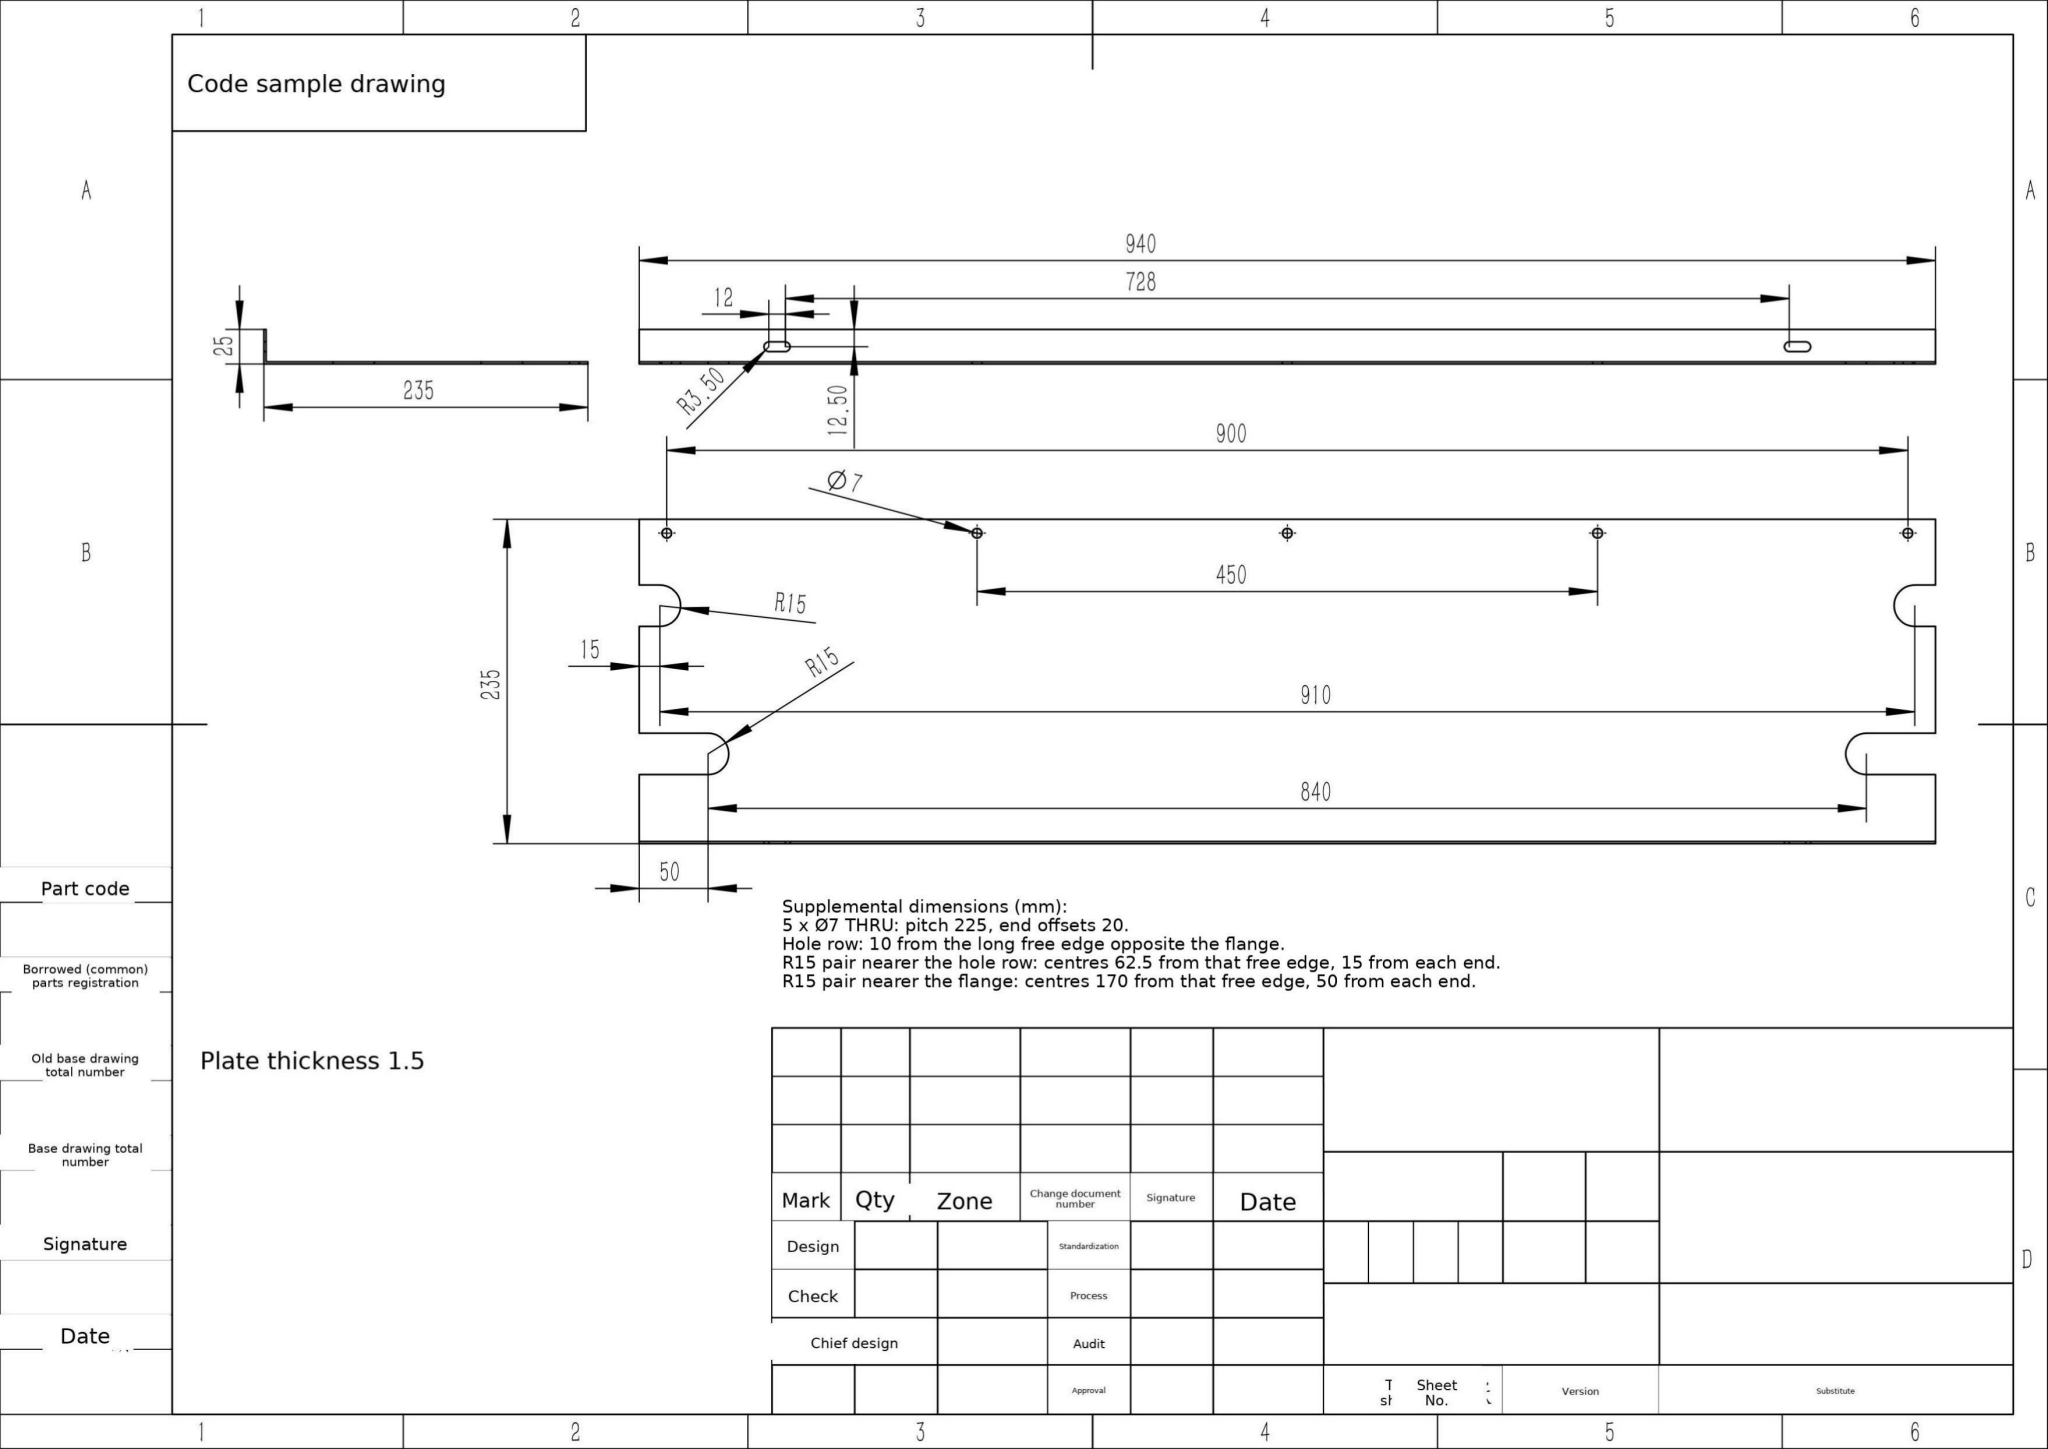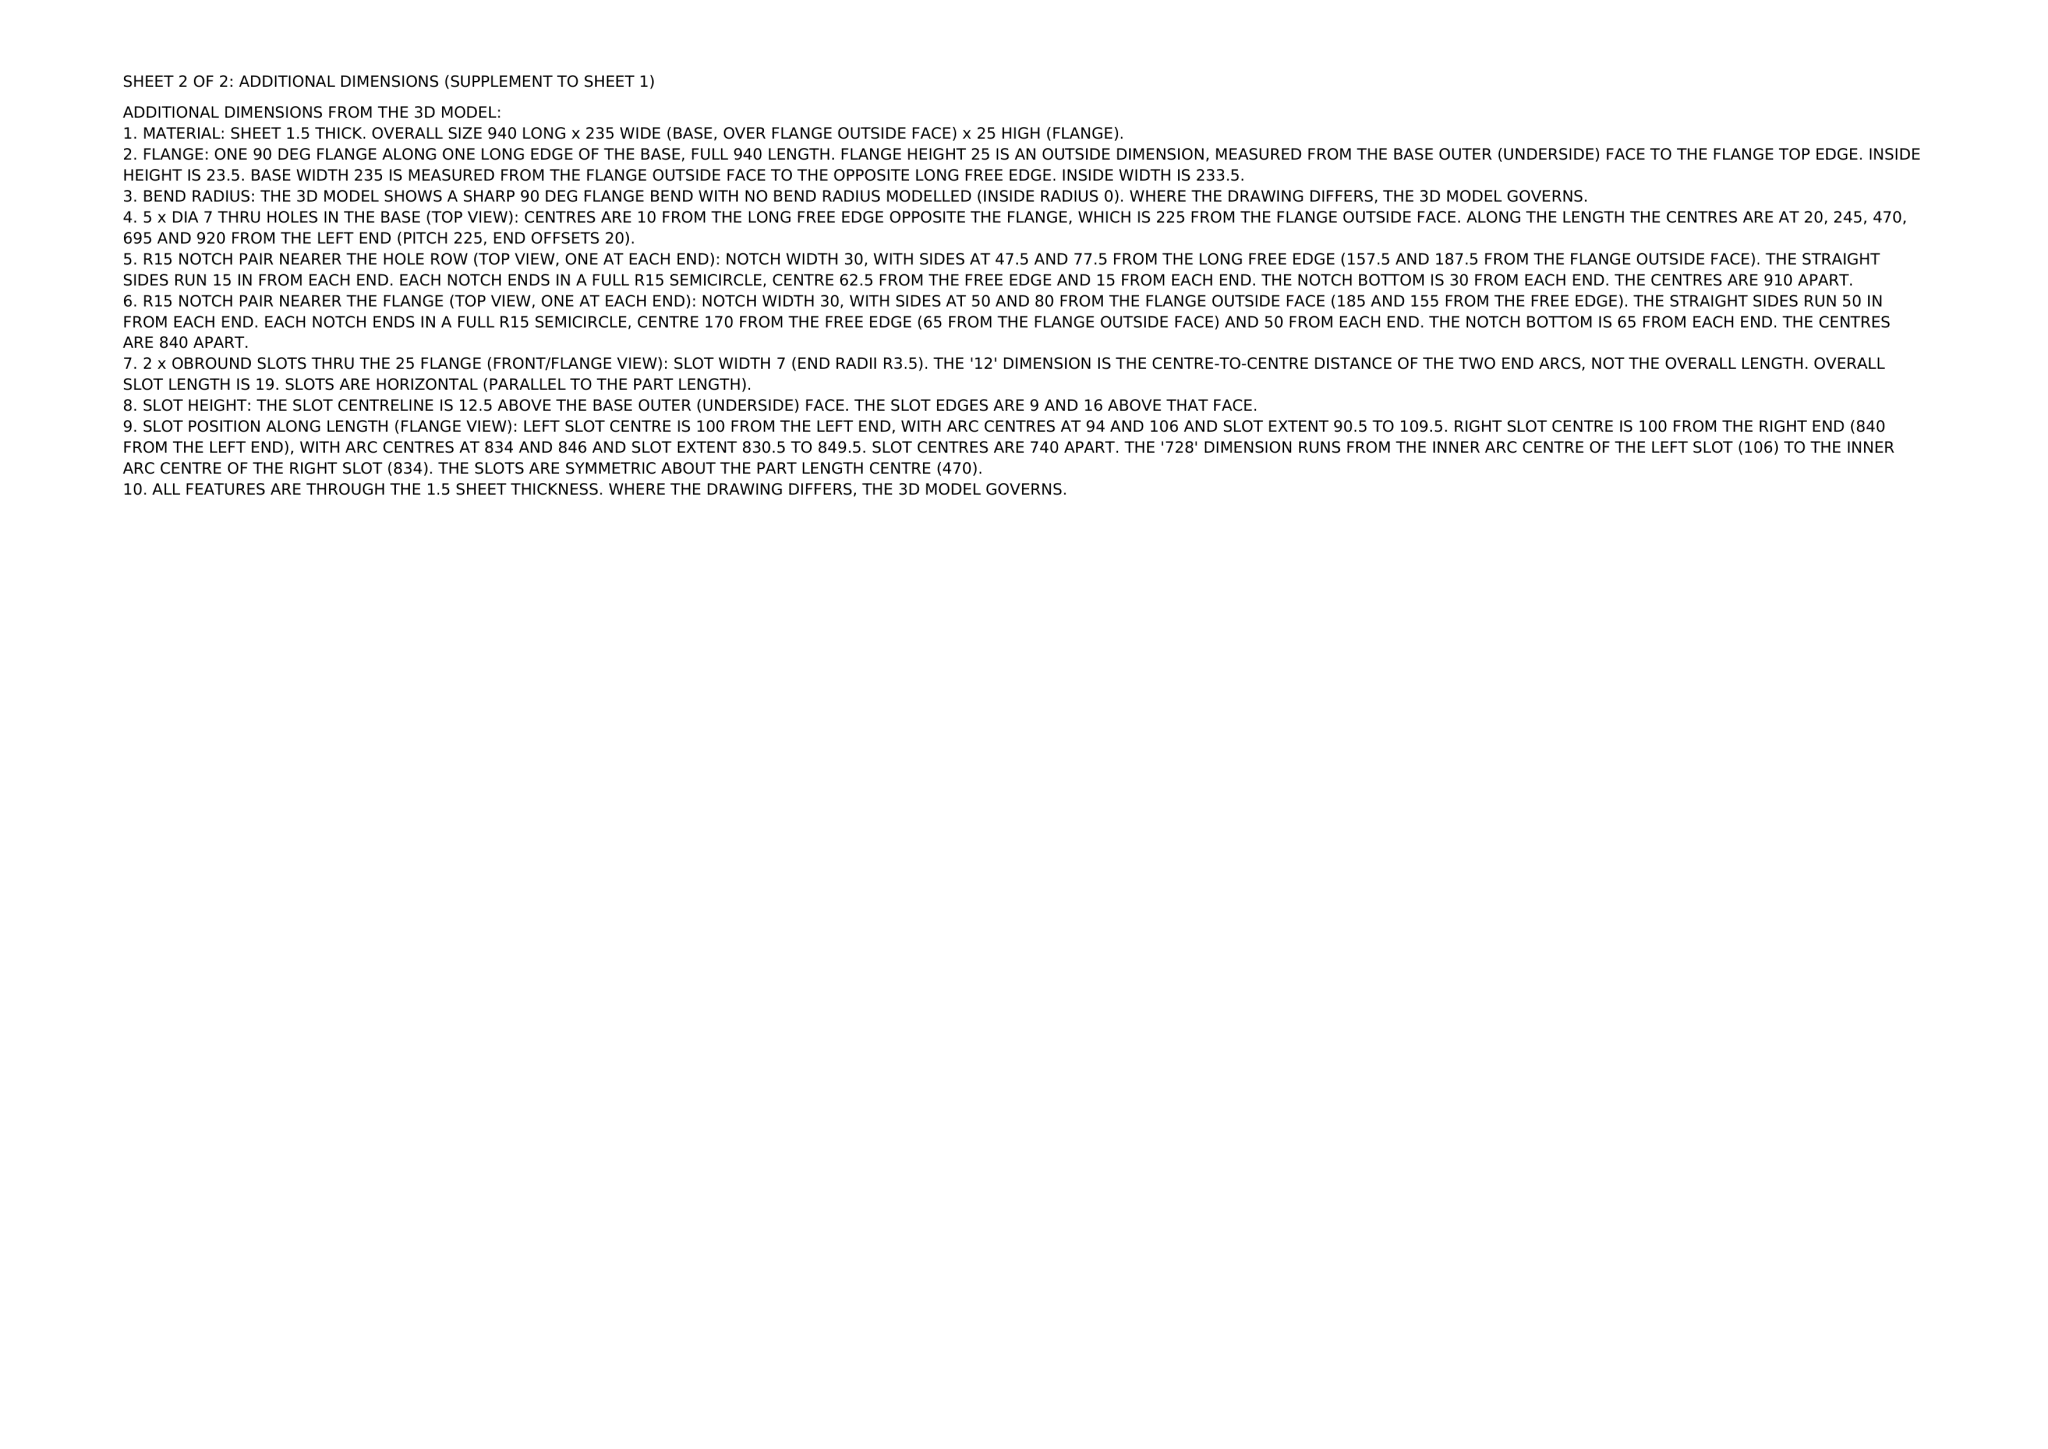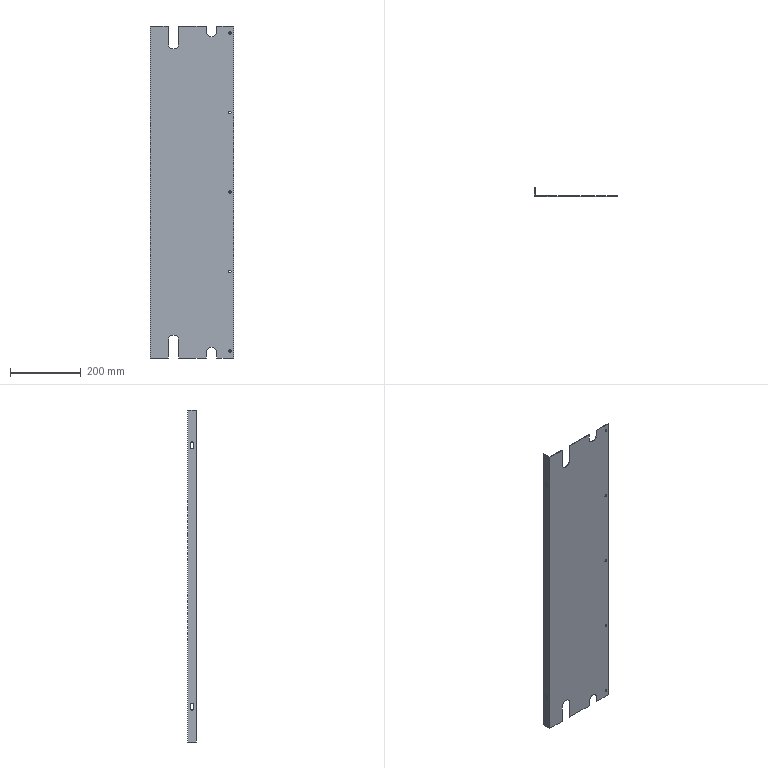Part | NX | mm | Notched Rectangular Panel Plate 940mm | 1 solid | 42 faces | box 235 x 25 x 940 mm | volume 355858 mm3 | plane 24 | cylinder 18 | commonest cylinder face diameters 7 x14 30 x4